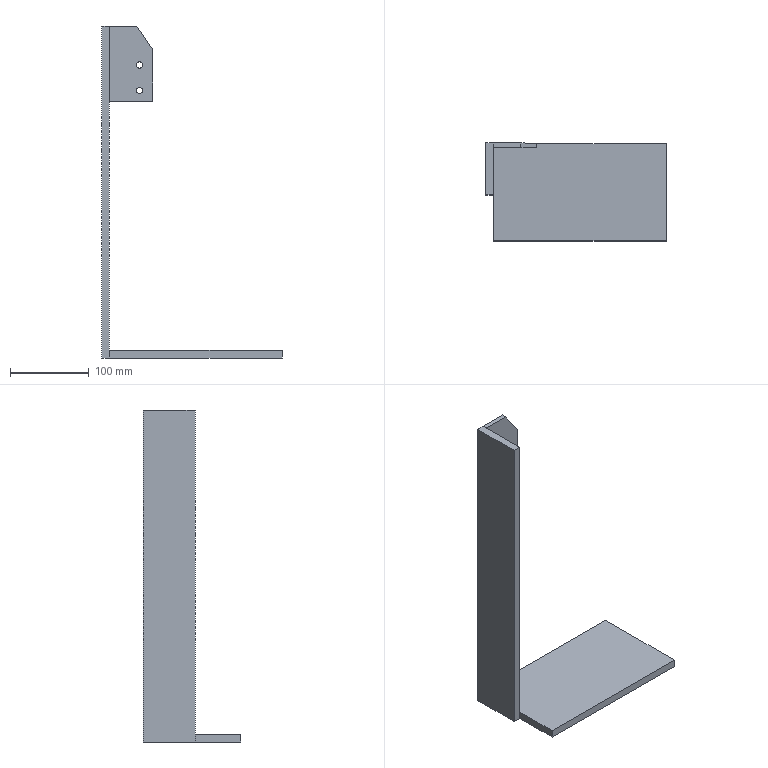Component | NX | VALVE_BODY_MOUNT | 3 solids | 21 faces | volume 580875 mm3 | plane 19 | cylinder 2 | commonest cylinder face diameters 8 x2